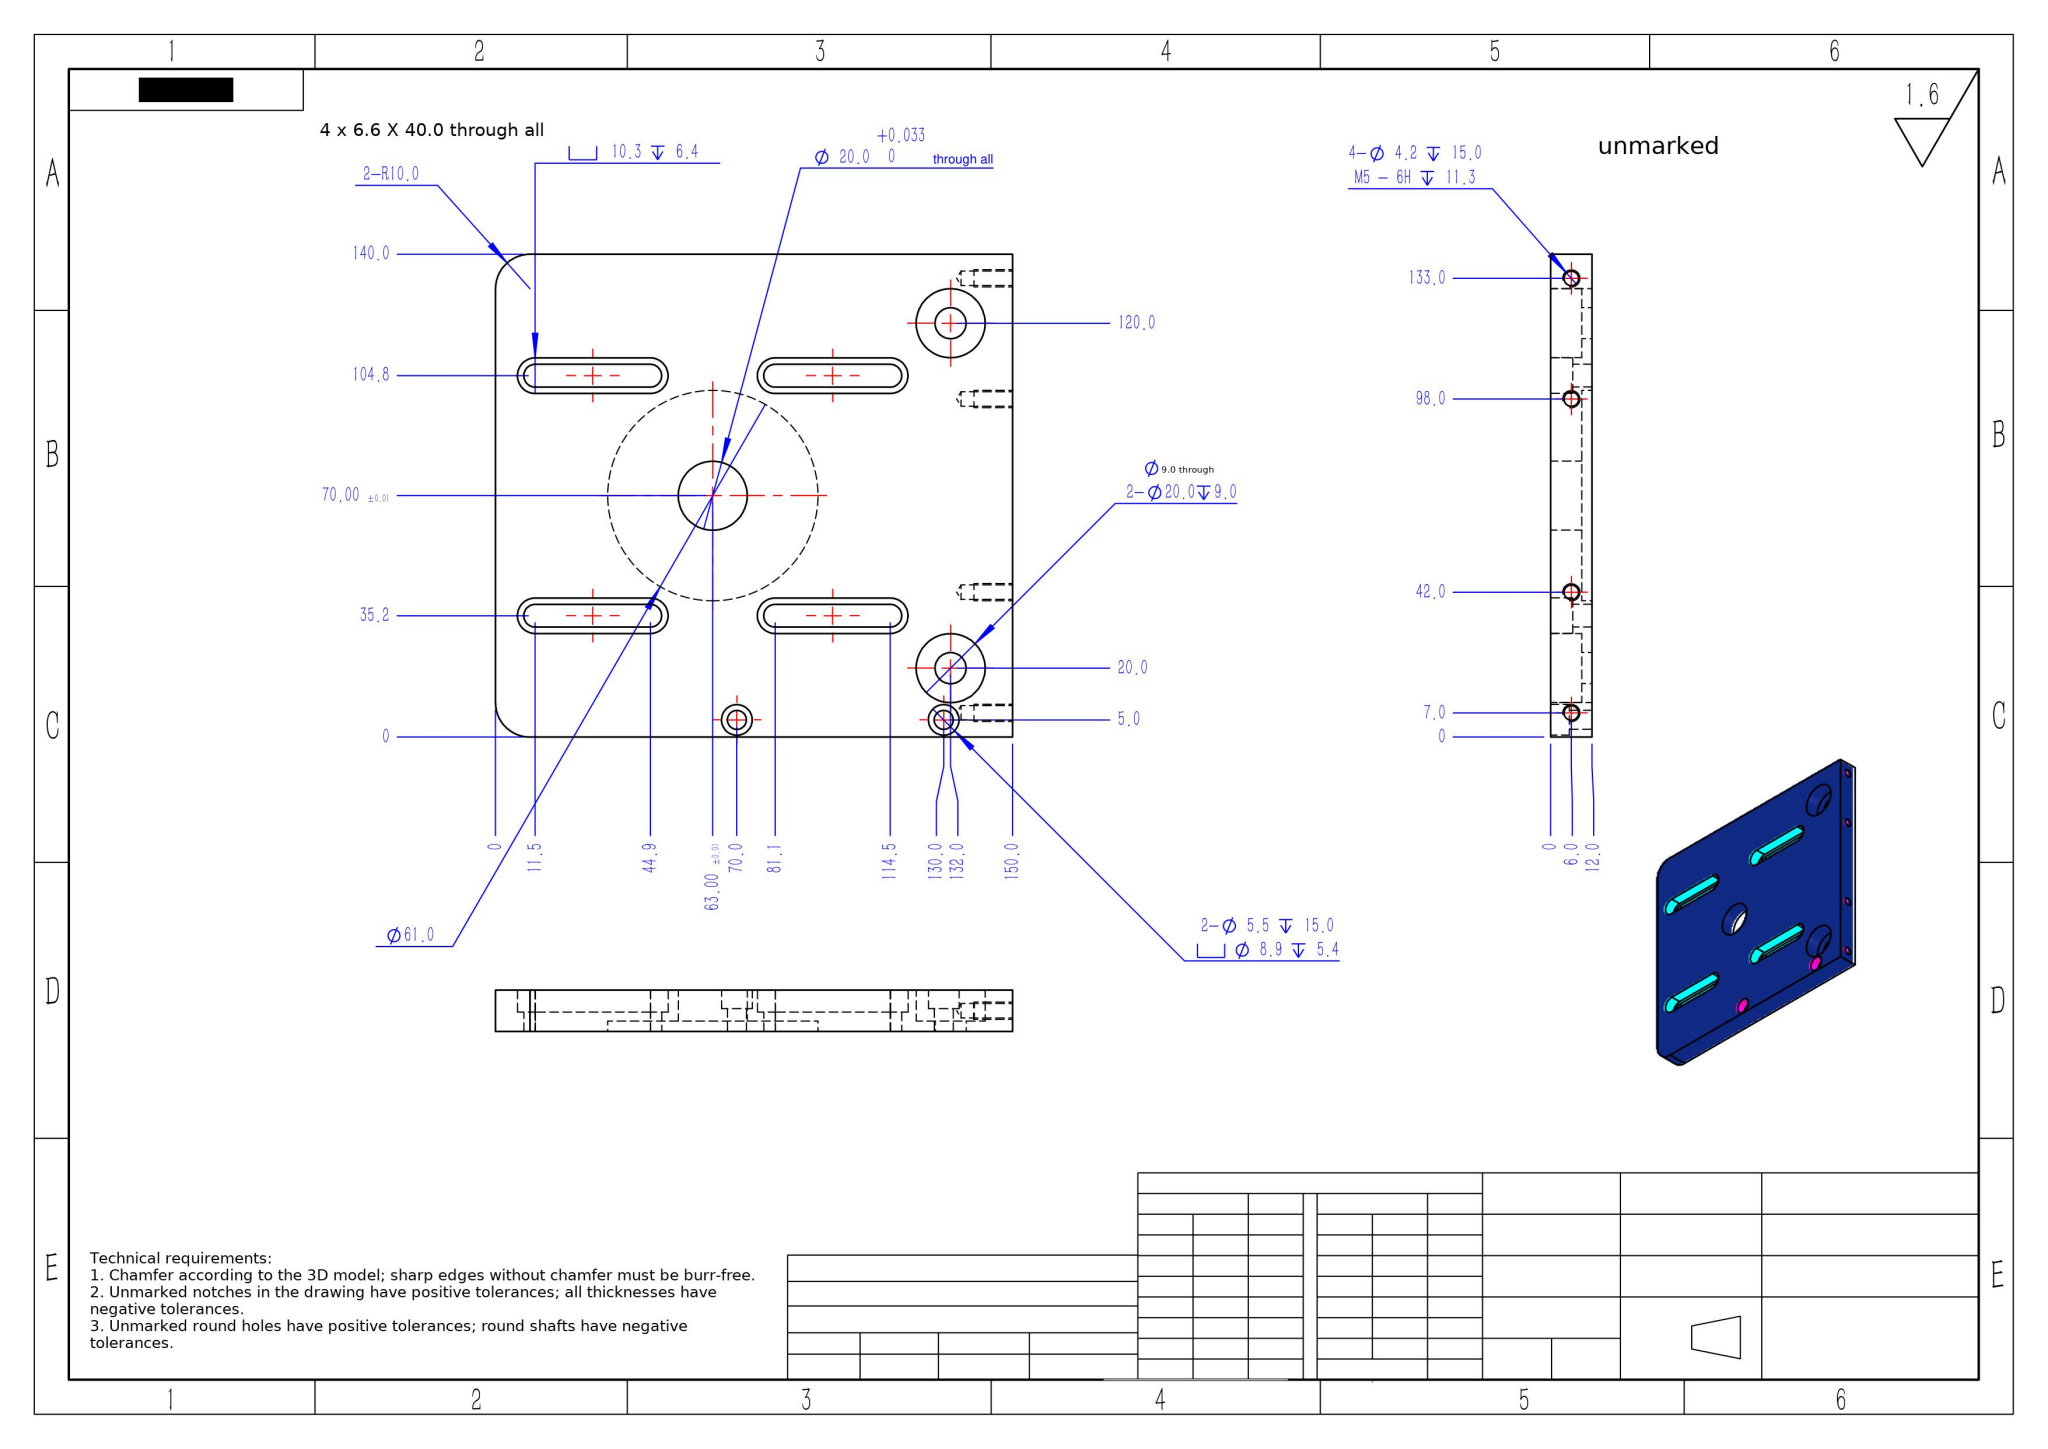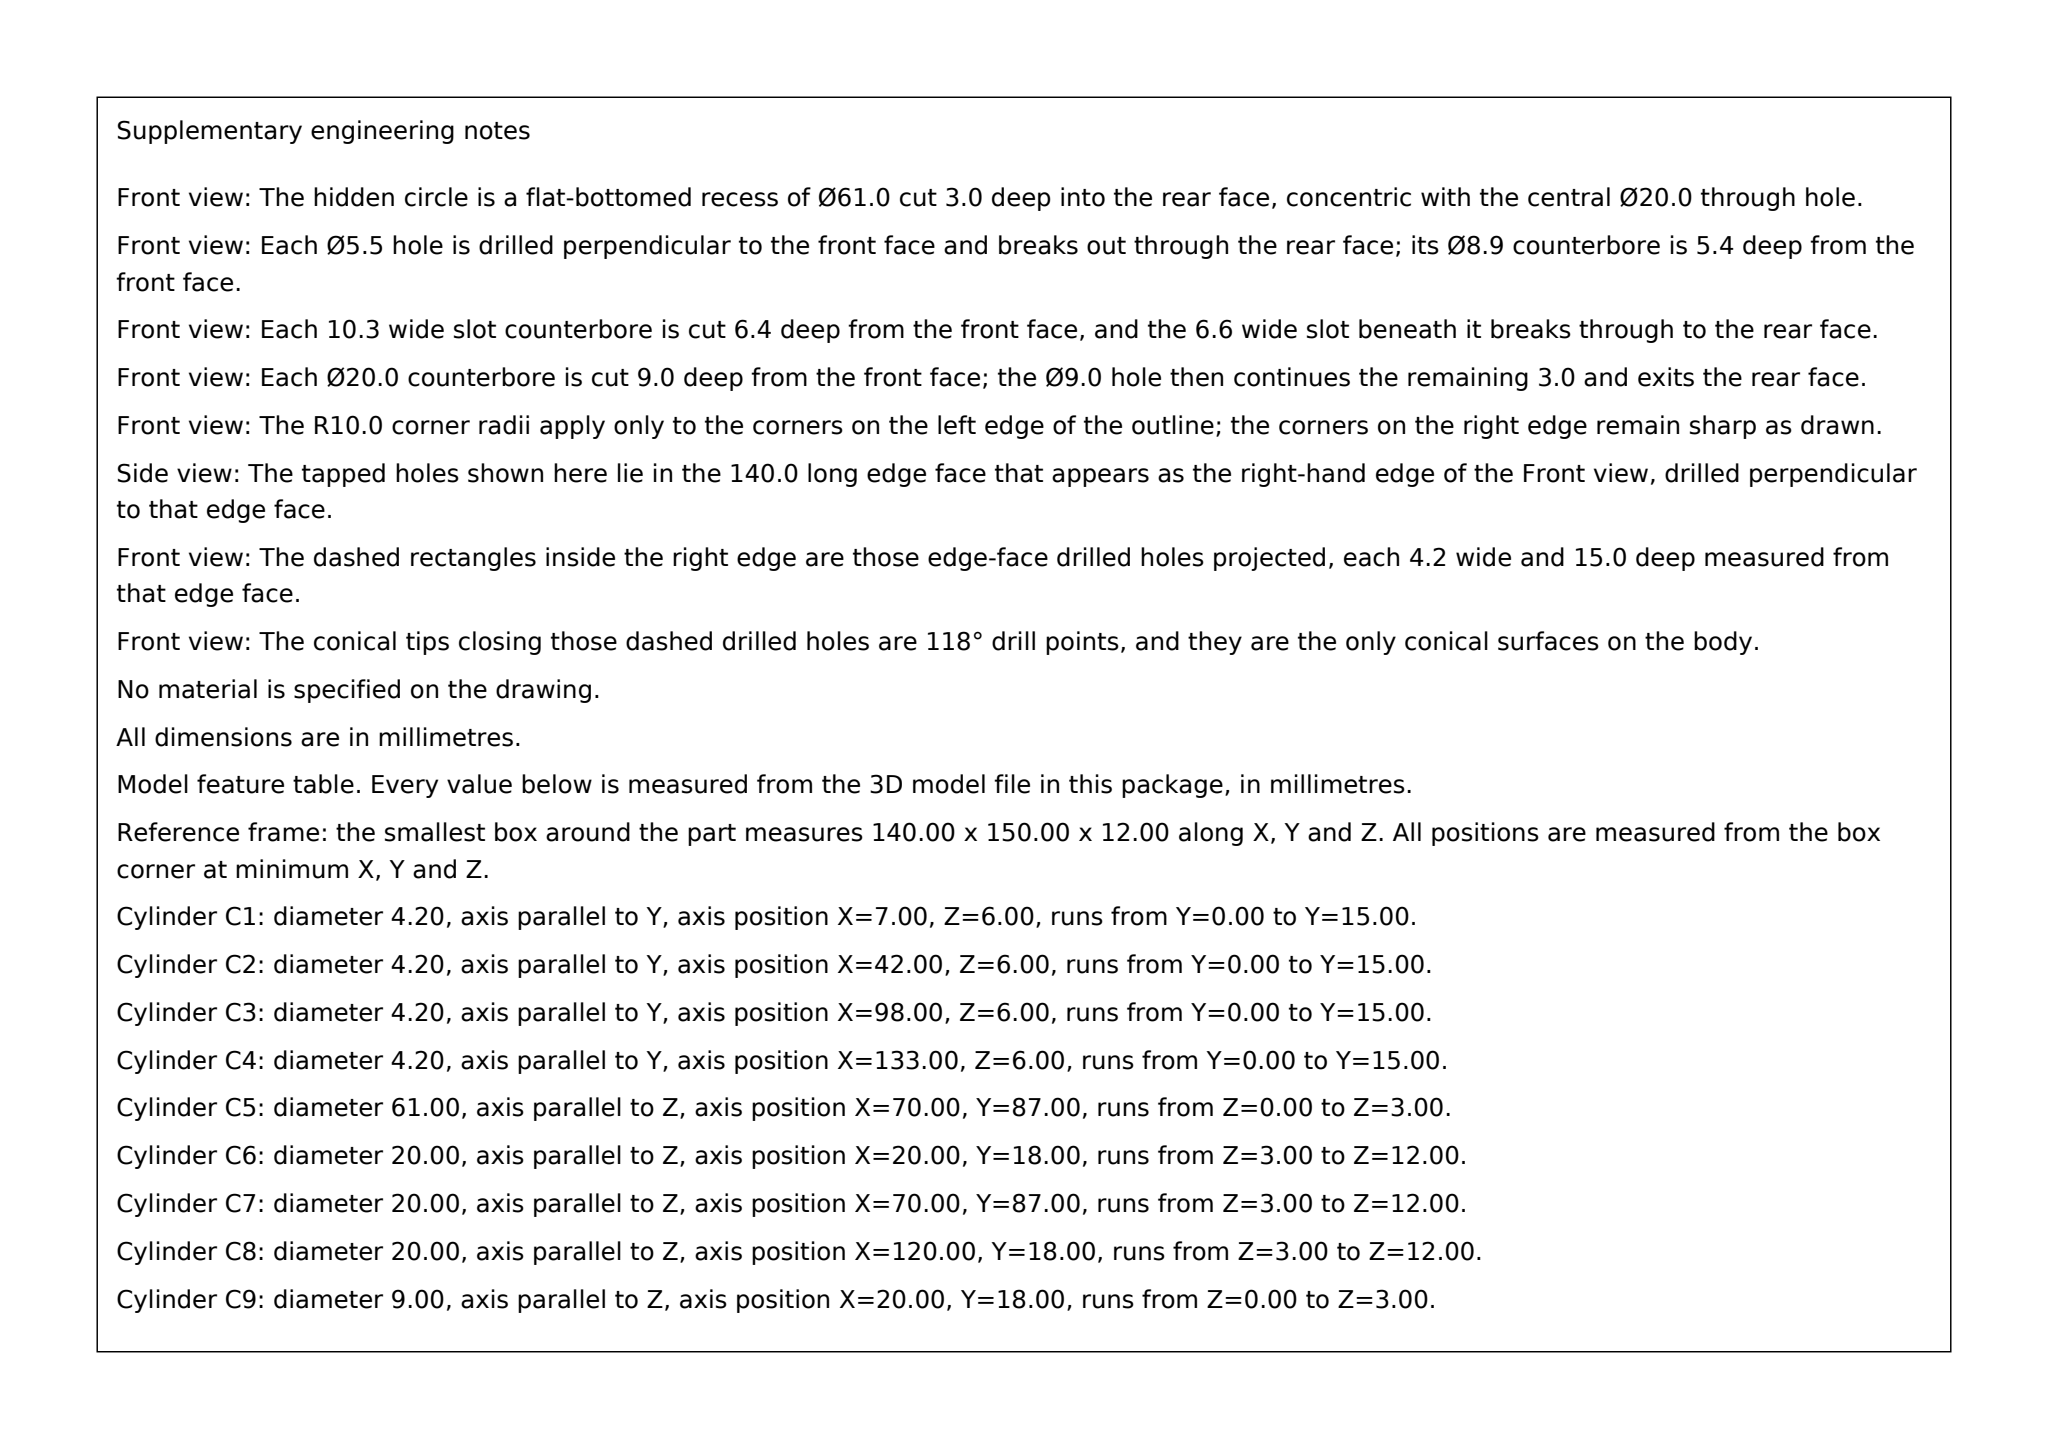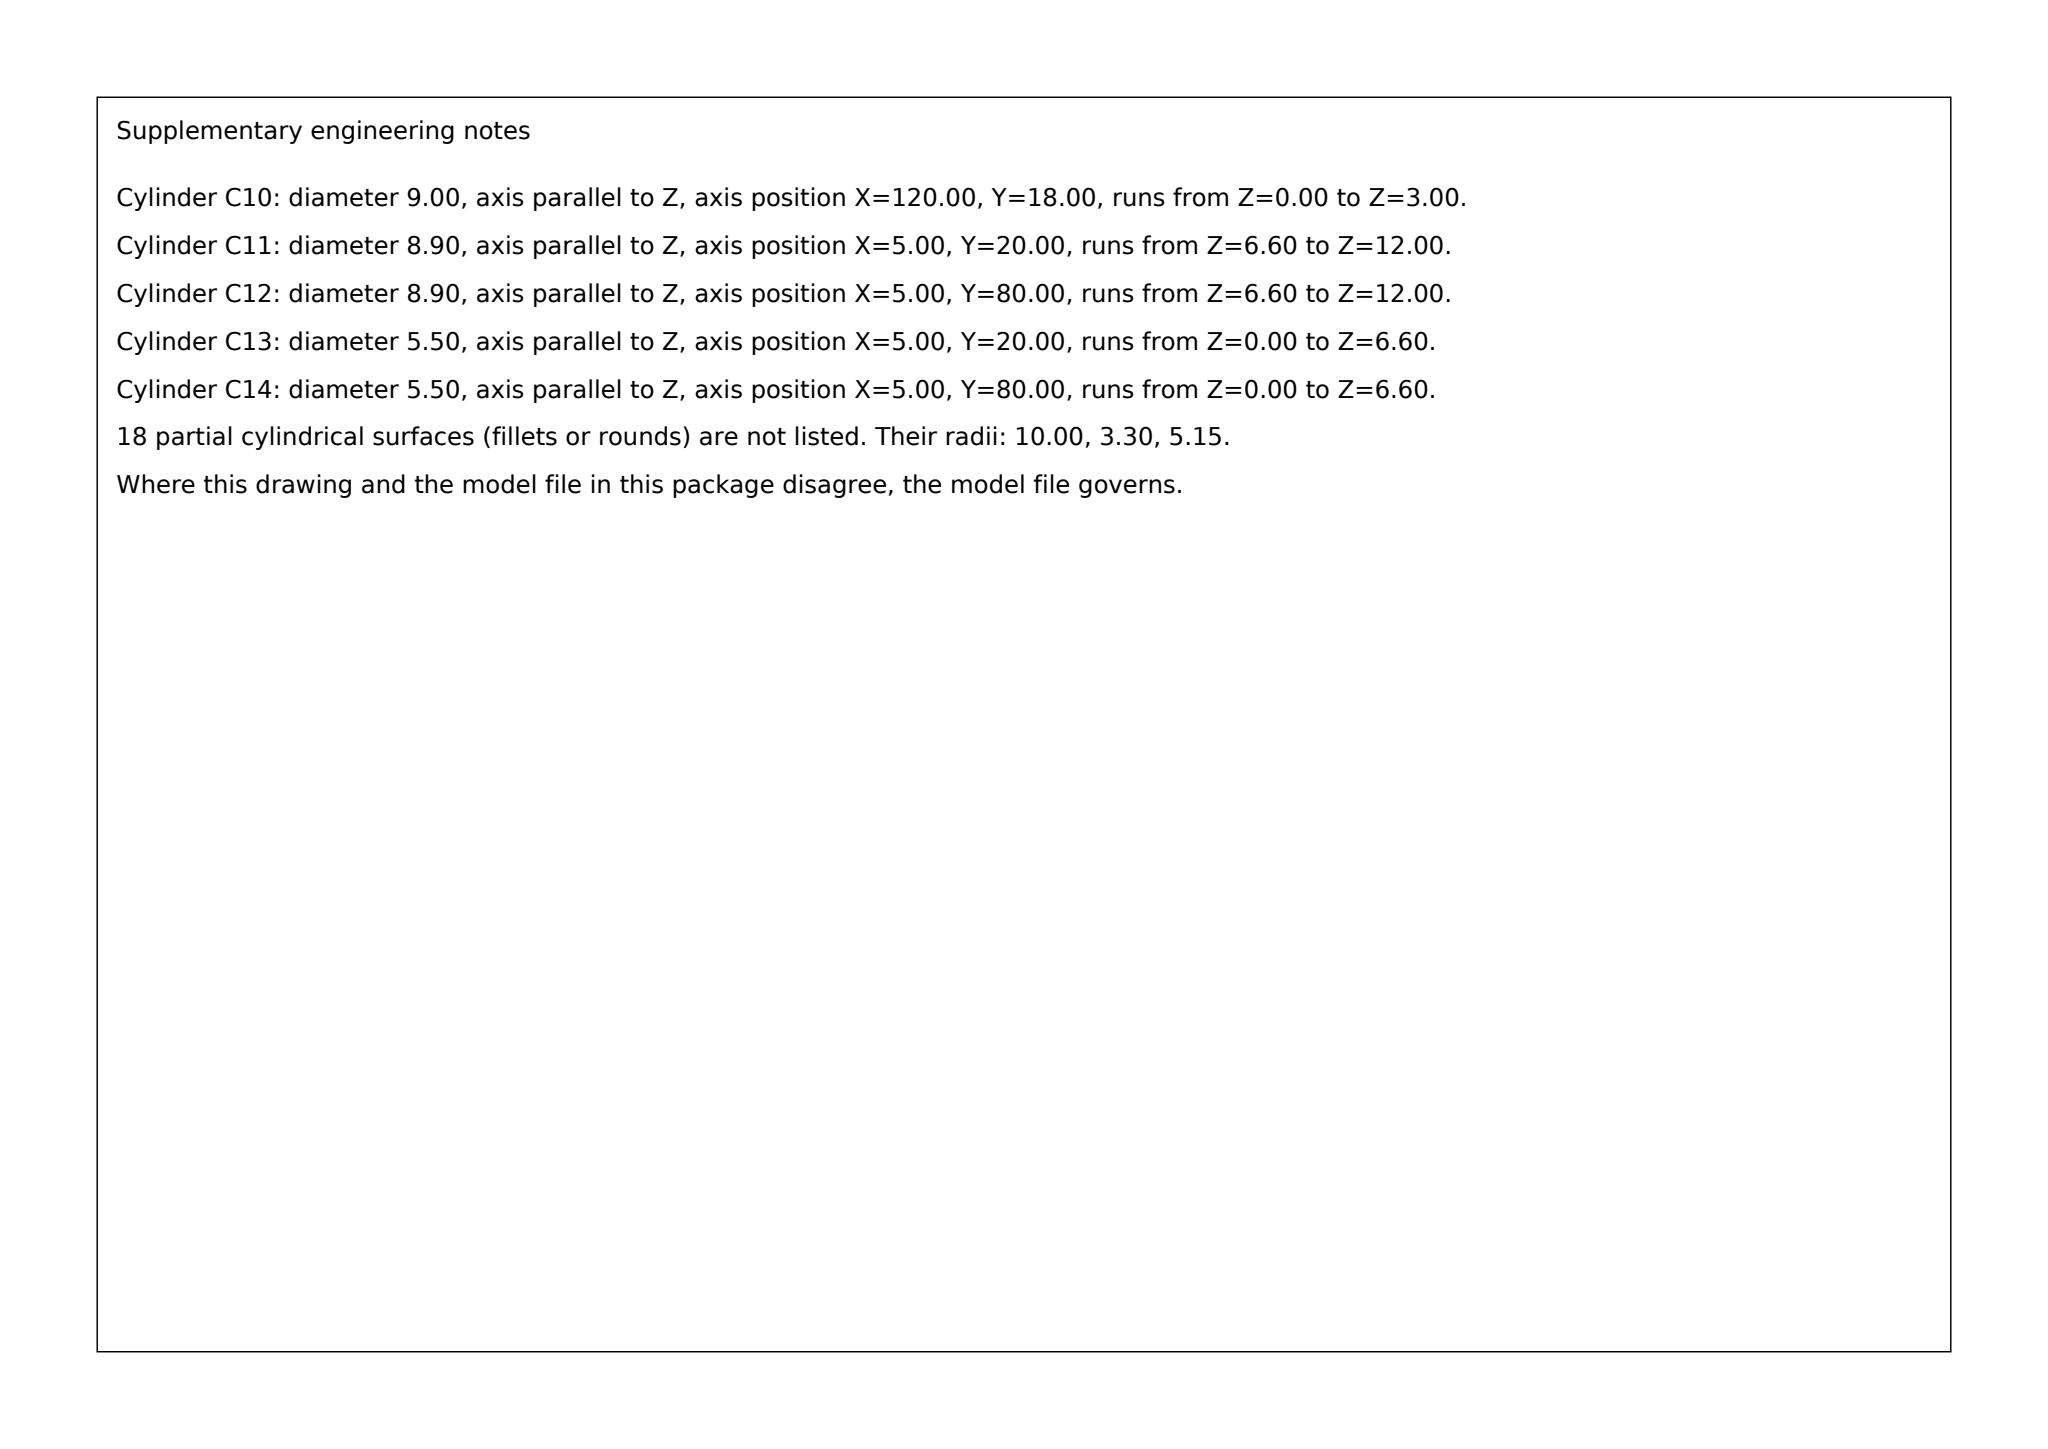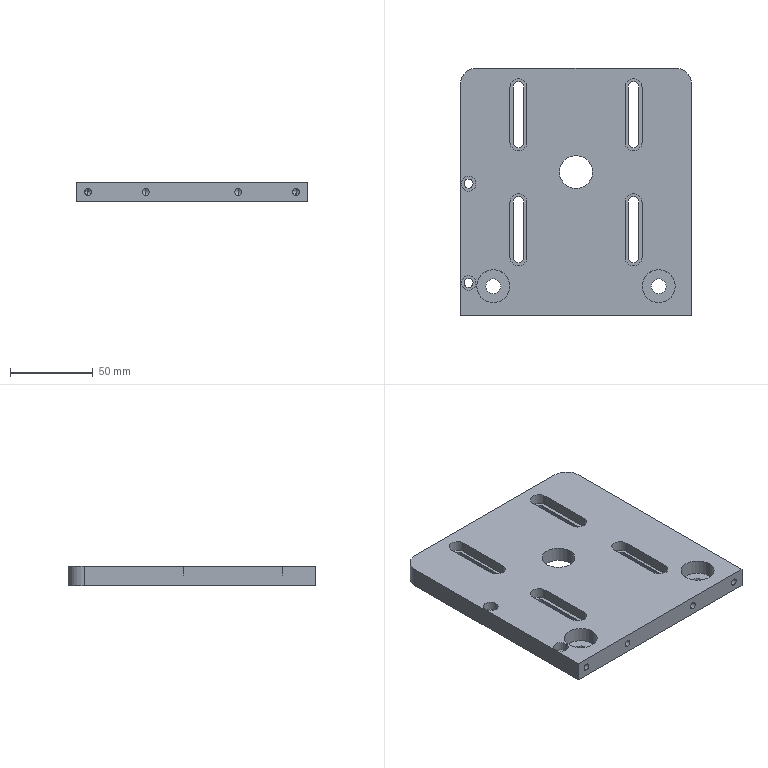Part | SolidWorks | mm | 1 solid | 85 faces | box 140 x 150 x 12 mm | volume 215369 mm3 | cylinder 46 | plane 31 | cone 8 | commonest cylinder face diameters 4.2 x8 20 x8 6.6 x8 10.3 x8 8.9 x4 5.5 x4 9 x4 61 x2